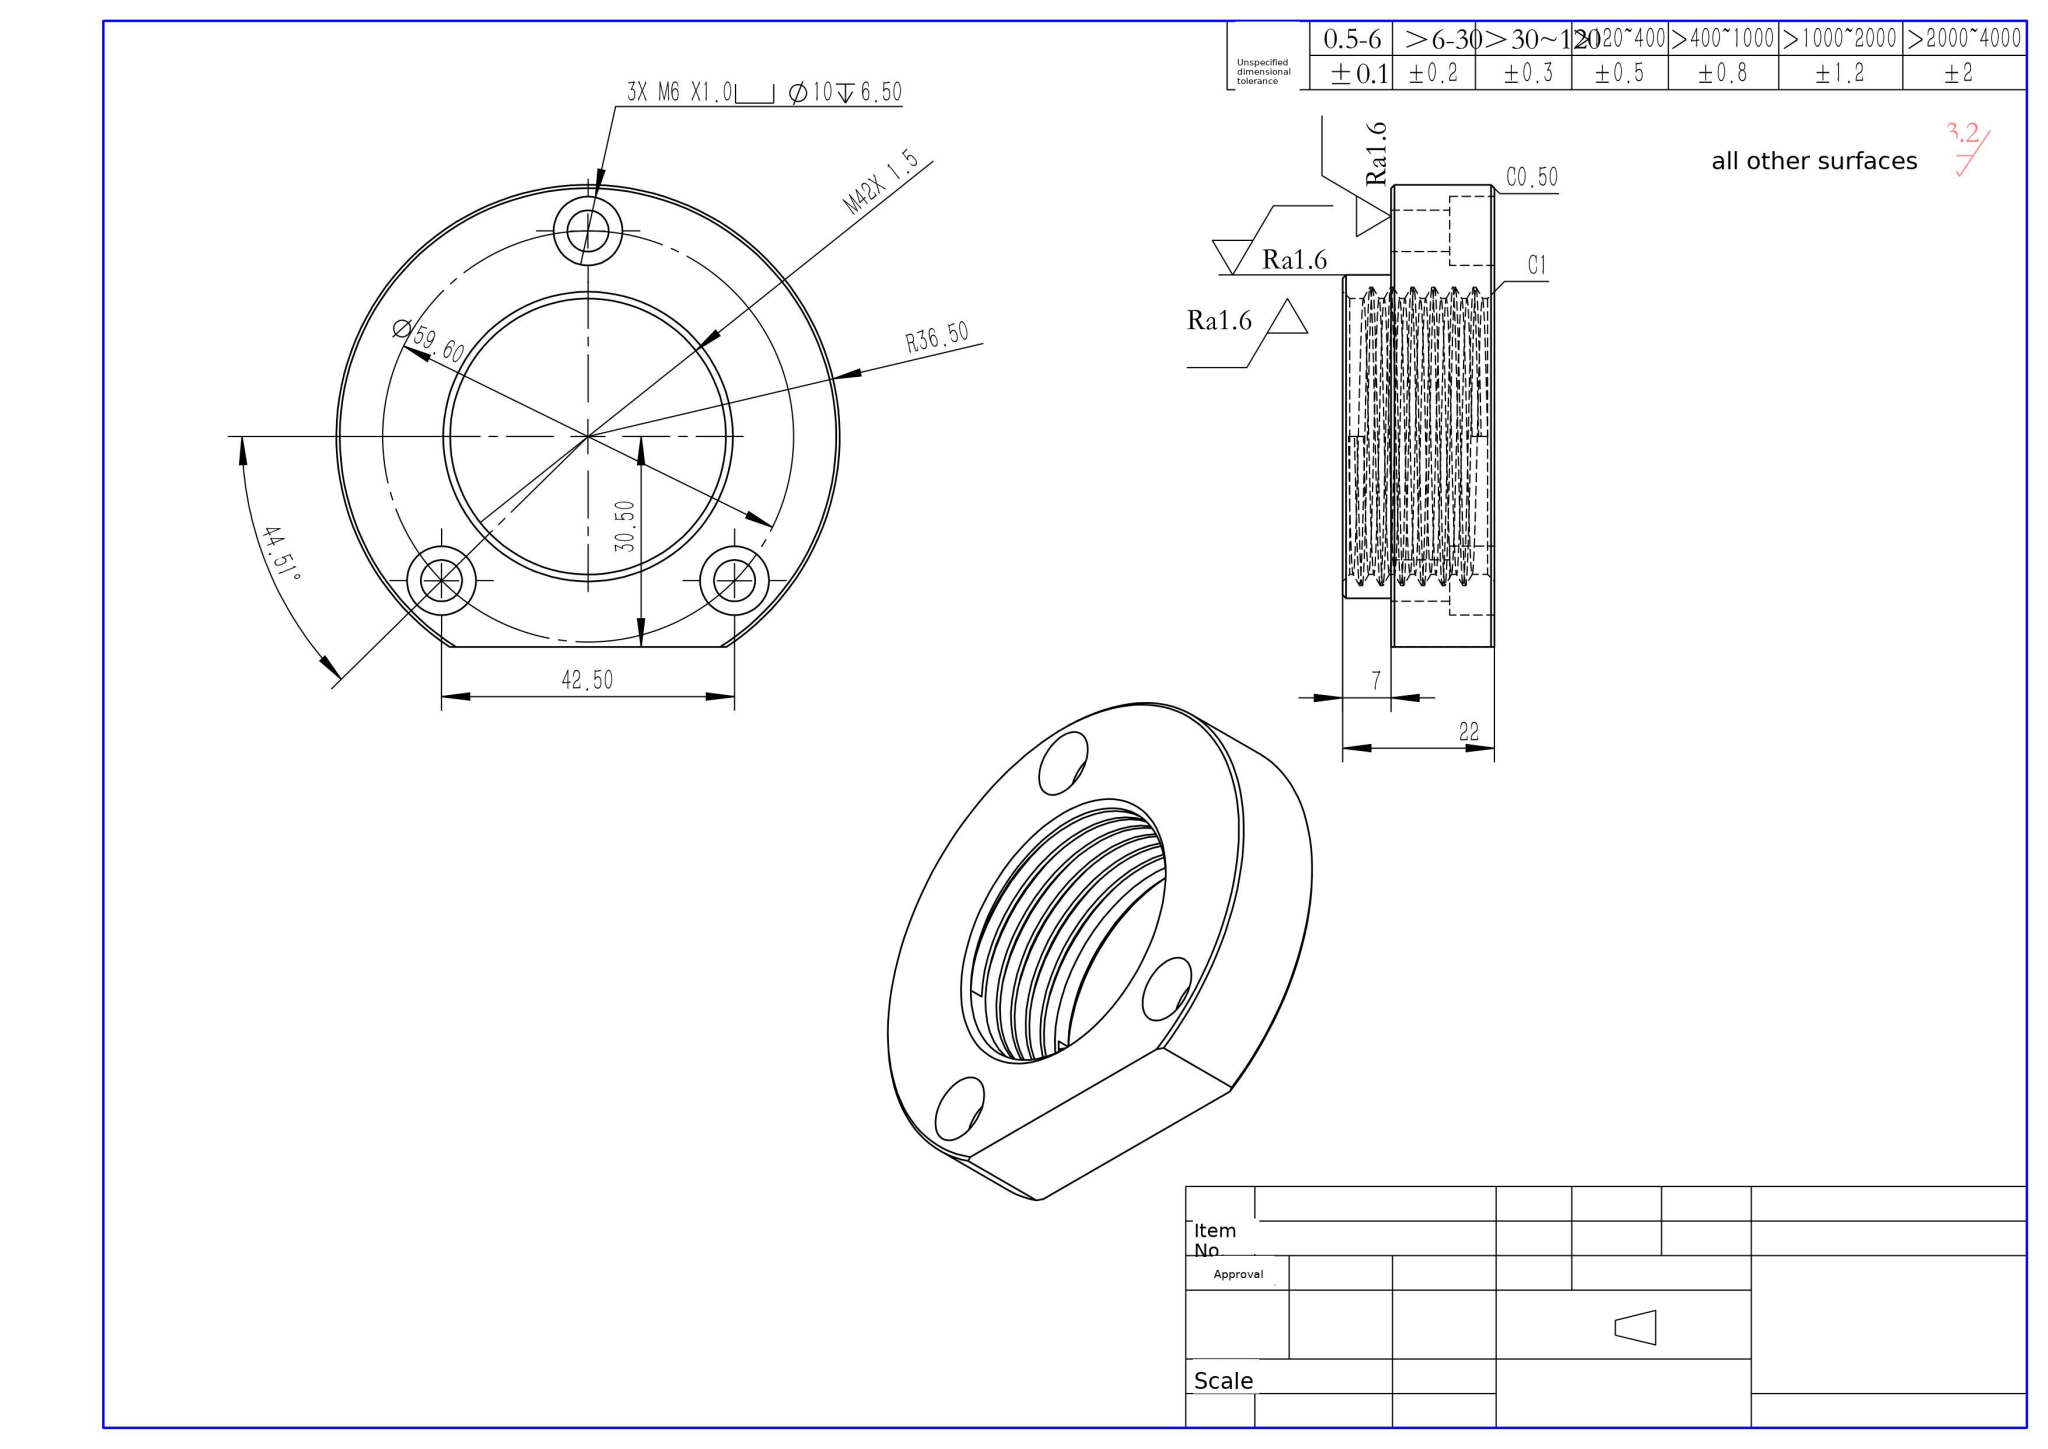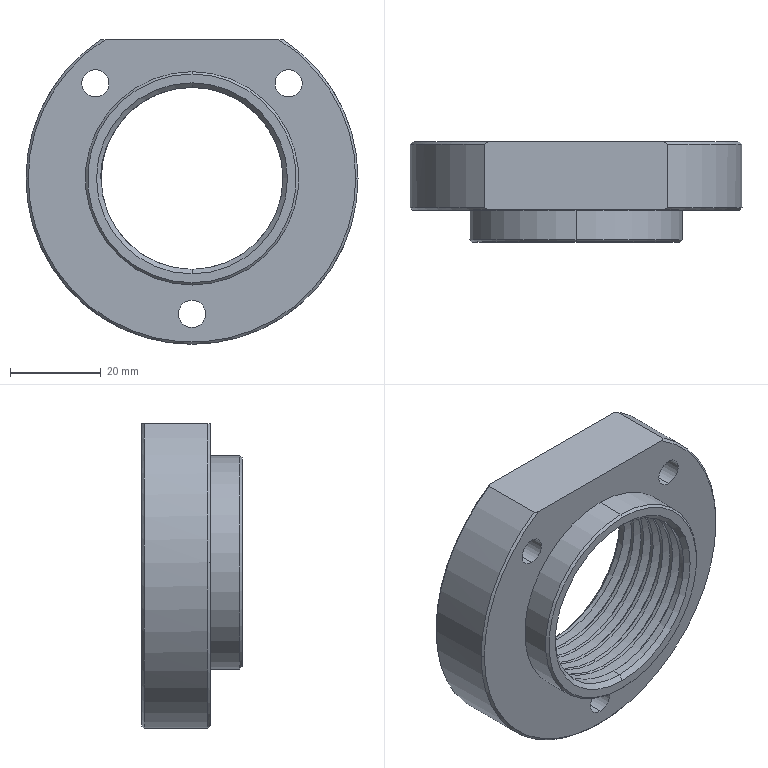Part | SolidWorks | mm | 1 solid | 53 faces | box 73 x 22 x 67 mm | volume 40683 mm3 | cylinder 30 | cone 11 | plane 9 | spline 3 | commonest cylinder face diameters 40 x15 6 x6 10 x6 46.9 x2 73 x1